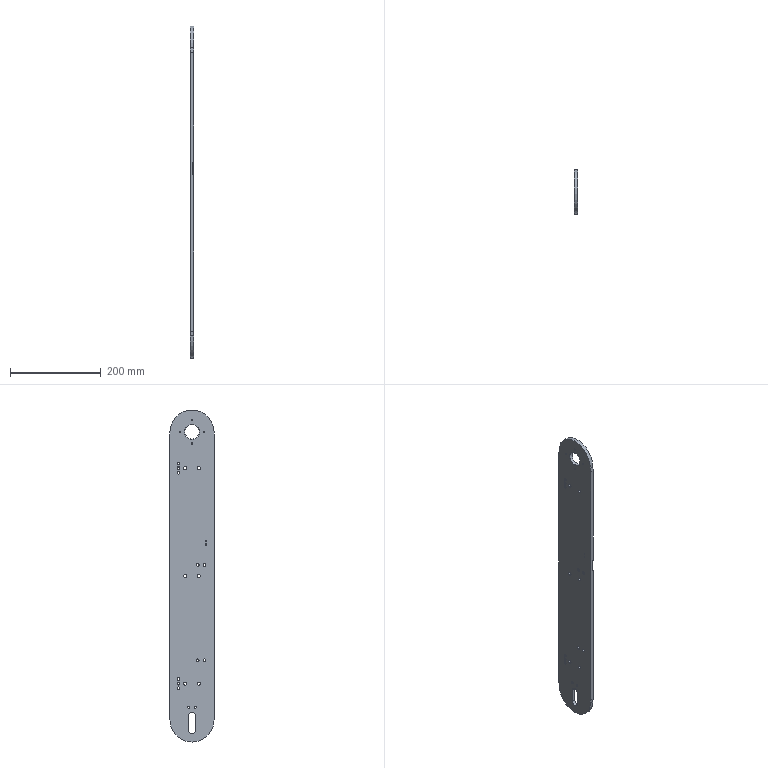Component | SolidWorks | ChainPartInnerSidePlate-1 | 1 solid | 84 faces | box 8 x 99 x 732 mm | volume 543846 mm3 | cylinder 58 | plane 14 | cone 12 | commonest cylinder face diameters 6 x16 7 x12 5 x8 3.3 x8 3 x4 97 x3 16 x3 32 x2
build123d program:
from build123d import *

# Parameters (mm, degrees)
BOSS_EXTRUDE1_DEPTH = 4
SKETCH3_R           = 16
CUT_EXTRUDE2_DEPTH  = 371.41
CUT_EXTRUDE3_DEPTH  = 10
M4_TAPPED_HOLE1_D   = 3.3
CHAMFER1_SIZE       = 0.5
SKETCH7_R           = 3.5
CUT_EXTRUDE4_DEPTH  = 10
CUT_EXTRUDE6_DEPTH  = 371.41
M5_TAPPED_HOLE2_D   = 5
M6_TAPPED_HOLE1_D   = 6
M6_TAPPED_HOLE2_D   = 6
SKETCH31_W          = 27
SKETCH31_H          = 27
CUT_EXTRUDE8_DEPTH  = 2
FILLET1_R           = 4
M3_TAPPED_HOLE1_D   = 3
SKETCH32_R          = 2.5
CUT_EXTRUDE9_DEPTH  = 370.419
CHAMFER2_SIZE       = 0.5


with BuildPart() as part:
    # Sketch1 → Boss-Extrude1 (new, symmetric)
    with BuildSketch(Plane.XY):
        with BuildLine():
            Line((-317.5, 49.5), (317.5, 49.5))
            ThreePointArc((317.5, 49.5), (367, 0), (317.5, -49.5))
            Line((317.5, -49.5), (-317.5, -49.5))
            ThreePointArc((-317.5, -49.5), (-367, 0), (-317.5, 49.5))
        make_face()
    extrude(amount=BOSS_EXTRUDE1_DEPTH, both=True)

    # Sketch3 → Cut-Extrude2 (cut, through all)
    with BuildSketch(Plane.XY.offset(4)):
        with Locations((-317.5, 0)):
            Circle(SKETCH3_R)
    extrude(amount=-CUT_EXTRUDE2_DEPTH, mode=Mode.SUBTRACT)

    # Sketch4 → Cut-Extrude3 (cut)
    with BuildSketch(Plane.XY.offset(4)):
        with BuildLine():
            Line((309.5, 8), (339.5, 8))
            ThreePointArc((339.5, 8), (347.5, 0), (339.5, -8))
            Line((339.5, -8), (309.5, -8))
            ThreePointArc((309.5, -8), (301.5, 0), (309.5, 8))
        make_face()
    extrude(amount=-CUT_EXTRUDE3_DEPTH, mode=Mode.SUBTRACT)

    # M4 Tapped Hole1 (through all)
    with Locations(Plane(origin=(0, 0, -4), x_dir=(-1, 0, 0), z_dir=(0, 0, -1))):
        with Locations((317.5, 26), (291.5, 0), (317.5, -26), (343.5, 0)):
            Hole(M4_TAPPED_HOLE1_D / 2)

    # Chamfer1
    chamfer1_edges = [part.edges().sort_by_distance(p)[0] for p in [
        (-333.5, 0, -4),
        (-333.5, 0, 4),
    ]]
    chamfer(chamfer1_edges, length=CHAMFER1_SIZE)

    # Sketch7 → Cut-Extrude4 (cut)
    with BuildSketch(Plane(origin=(0, 0, -4), x_dir=(-1, 0, 0), z_dir=(0, 0, -1))):
        with Locations((237.5, 15)):
            Circle(SKETCH7_R)
        with Locations((237.5, -15)):
            Circle(SKETCH7_R)
        with Locations((-237.5, 15)):
            Circle(SKETCH7_R)
        with Locations((-237.5, -15)):
            Circle(SKETCH7_R)
        with Locations((0, 15)):
            Circle(SKETCH7_R)
        with Locations((0, -15)):
            Circle(SKETCH7_R)
    extrude(amount=-CUT_EXTRUDE4_DEPTH, mode=Mode.SUBTRACT)

    # Sketch13 → Cut-Extrude6 (cut, through all)
    with BuildSketch(Plane.XY.offset(4)):
        with BuildLine():
            Line((307.5, 49.5), (317.5, 48.5))
            ThreePointArc((317.5, 48.5), (366, 0), (317.5, -48.5))
            Line((317.5, -48.5), (307.5, -49.5))
            Line((307.5, -49.5), (317.5, -49.5))
            ThreePointArc((317.5, -49.5), (367, 0), (317.5, 49.5))
            Line((317.5, 49.5), (307.5, 49.5))
        make_face()
        with BuildLine():
            Line((-307.5, 49.5), (-317.5, 48.5))
            ThreePointArc((-317.5, 48.5), (-366, 0), (-317.5, -48.5))
            Line((-317.5, -48.5), (-307.5, -49.5))
            Line((-307.5, -49.5), (-317.5, -49.5))
            ThreePointArc((-317.5, -49.5), (-367, 0), (-317.5, 49.5))
            Line((-317.5, 49.5), (-307.5, 49.5))
        make_face()
    extrude(amount=-CUT_EXTRUDE6_DEPTH, mode=Mode.SUBTRACT)

    # M5 Tapped Hole2 (through all)
    with Locations(Plane.XY.offset(4)):
        with Locations((289.5, 7), (289.5, -7)):
            Hole(M5_TAPPED_HOLE2_D / 2)

    # M6 Tapped Hole1 (through all)
    with Locations(Plane(origin=(0, 0, -4), x_dir=(-1, 0, 0), z_dir=(0, 0, -1))):
        with Locations((-247.5, 30), (-227.5, 30), (227.5, 30), (247.5, 30)):
            Hole(M6_TAPPED_HOLE1_D / 2)

    # M6 Tapped Hole2 (through all)
    with Locations(Plane(origin=(0, 0, -4), x_dir=(-1, 0, 0), z_dir=(0, 0, -1))):
        with Locations((-185.75, -27.5), (-185.75, -12.5), (24.25, -12.5), (24.25, -27.5)):
            Hole(M6_TAPPED_HOLE2_D / 2)

    # Sketch31 → Cut-Extrude8 (cut)
    with BuildSketch(Plane.XY.offset(4)):
        with Locations((-51.75, -36)):
            Rectangle(SKETCH31_W, SKETCH31_H)
    extrude(amount=-CUT_EXTRUDE8_DEPTH, mode=Mode.SUBTRACT)

    # Fillet1
    fillet1_edges = [part.edges().sort_by_distance(p)[0] for p in [
        (-65.25, -22.5, 3),
        (-38.25, -22.5, 3),
    ]]
    fillet(fillet1_edges, radius=FILLET1_R)

    # M3 Tapped Hole1 (through all)
    with Locations(Plane.XY.offset(4)):
        with Locations((-77.25, -30.5), (-69.25, -30.5)):
            Hole(M3_TAPPED_HOLE1_D / 2)

    # Sketch32 → Cut-Extrude9 (cut, through all)
    with BuildSketch(Plane(origin=(0, 0, -4), x_dir=(-1, 0, 0), z_dir=(0, 0, -1))):
        with Locations((-237.5, 30)):
            Circle(SKETCH32_R)
        with Locations((237.5, 30)):
            Circle(SKETCH32_R)
    extrude(amount=-CUT_EXTRUDE9_DEPTH, mode=Mode.SUBTRACT)

    # Chamfer2
    chamfer2_edges = [part.edges().sort_by_distance(p)[0] for p in [
        (240, 30, 4),
        (240, 30, -4),
        (-235, 30, 4),
        (-235, 30, -4),
    ]]
    chamfer(chamfer2_edges, length=CHAMFER2_SIZE)


solid = part.part

# Placed as in the assembly
solid = solid.moved(Location((131.637, -2.563, -352.804), (0, 90, 0)))